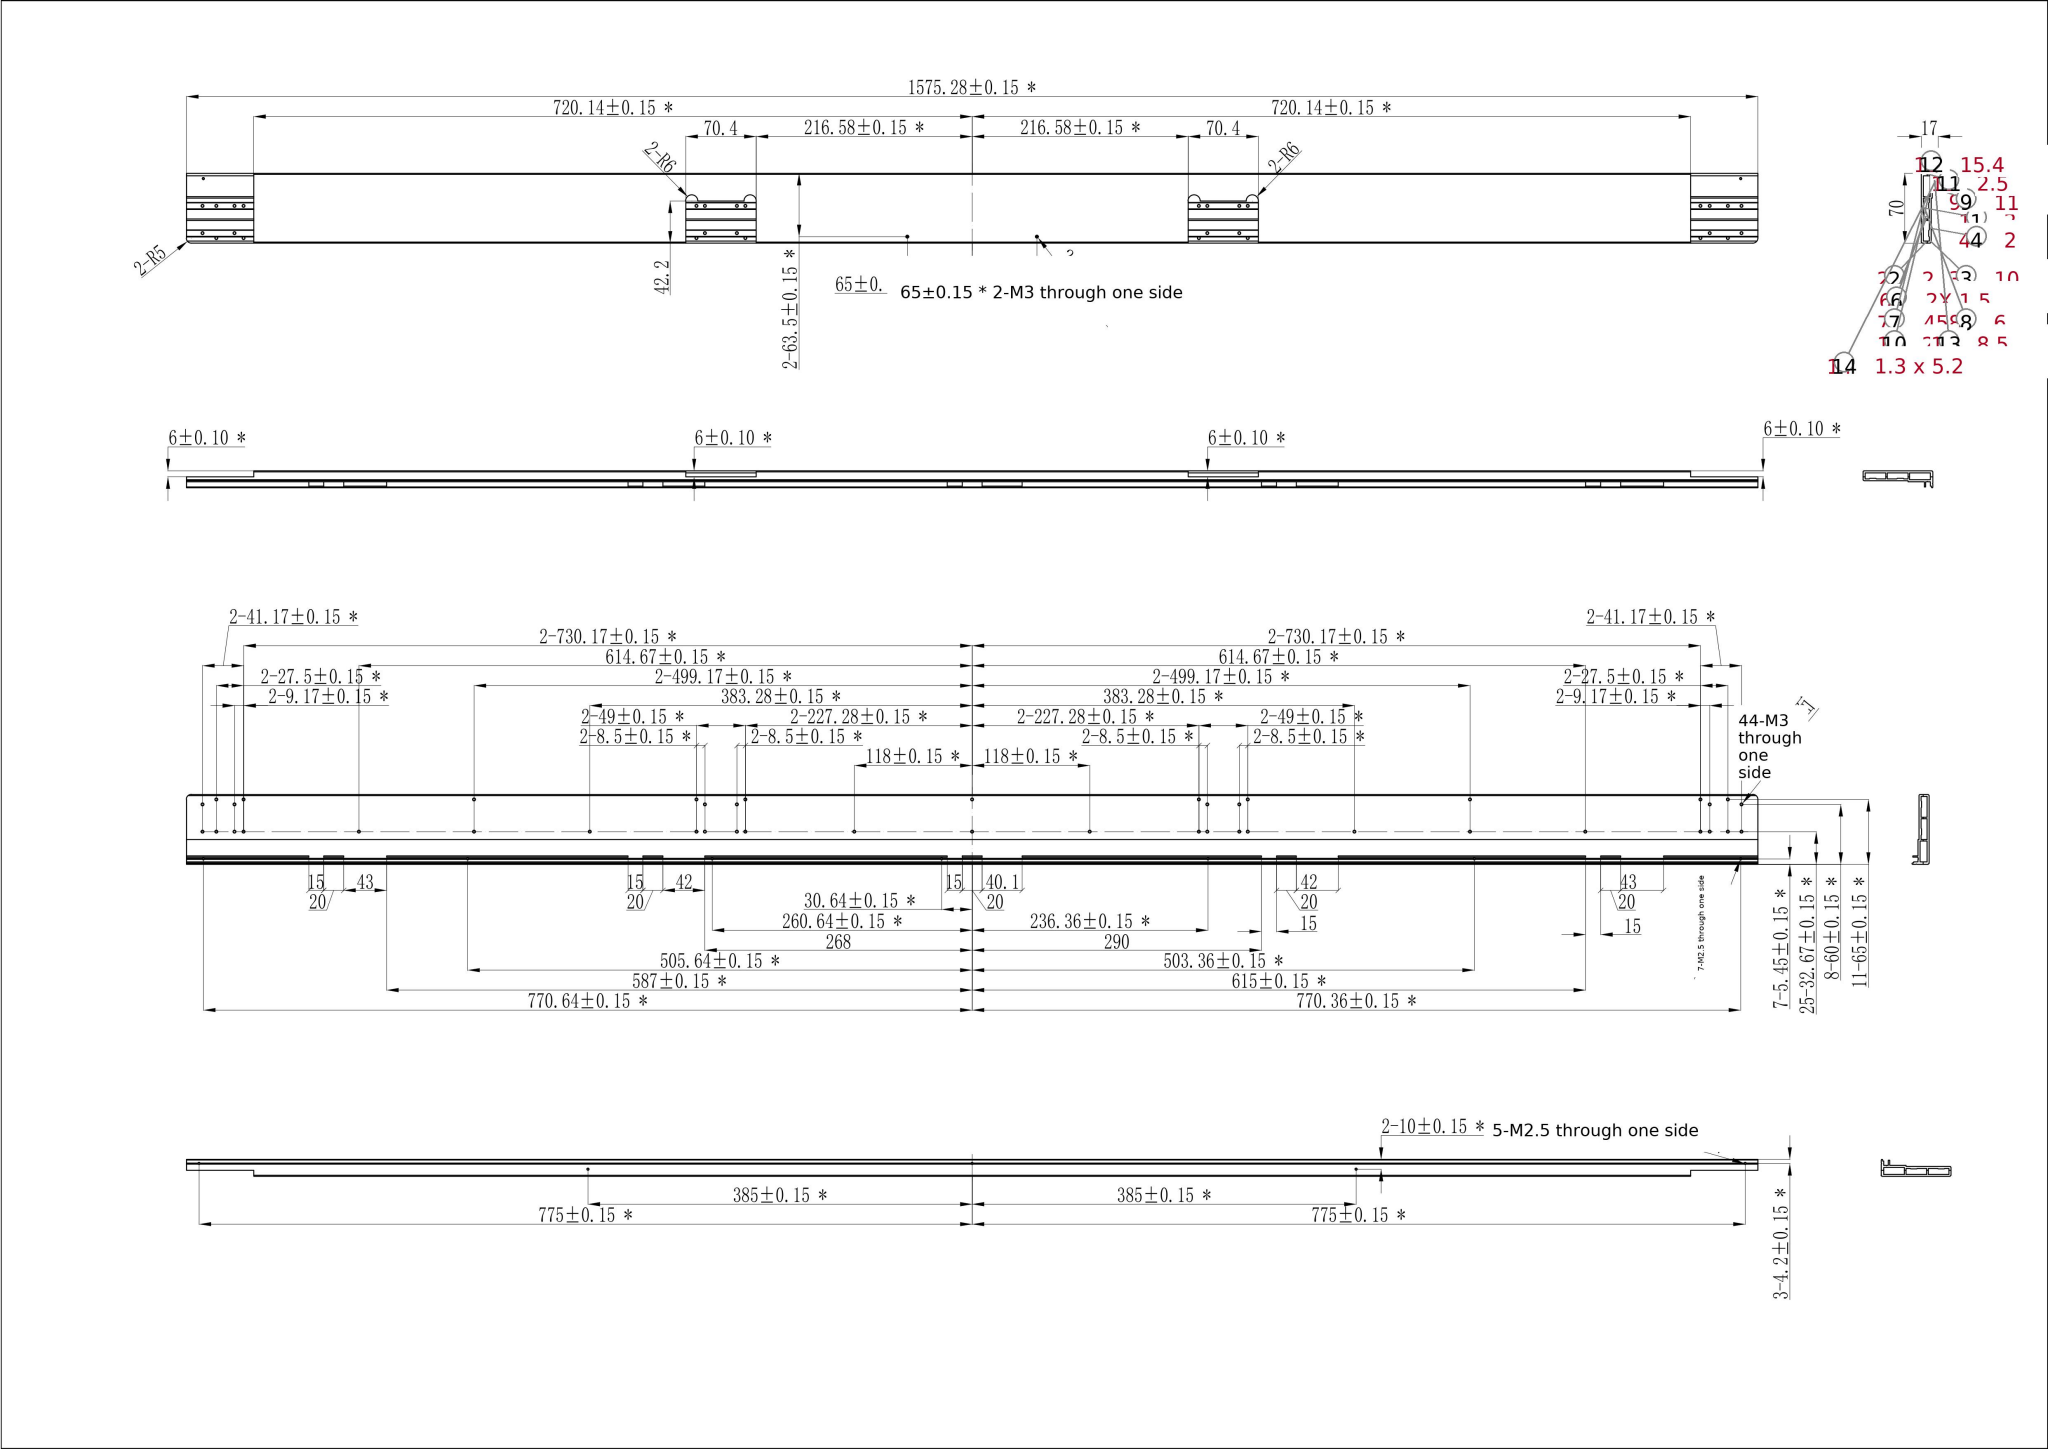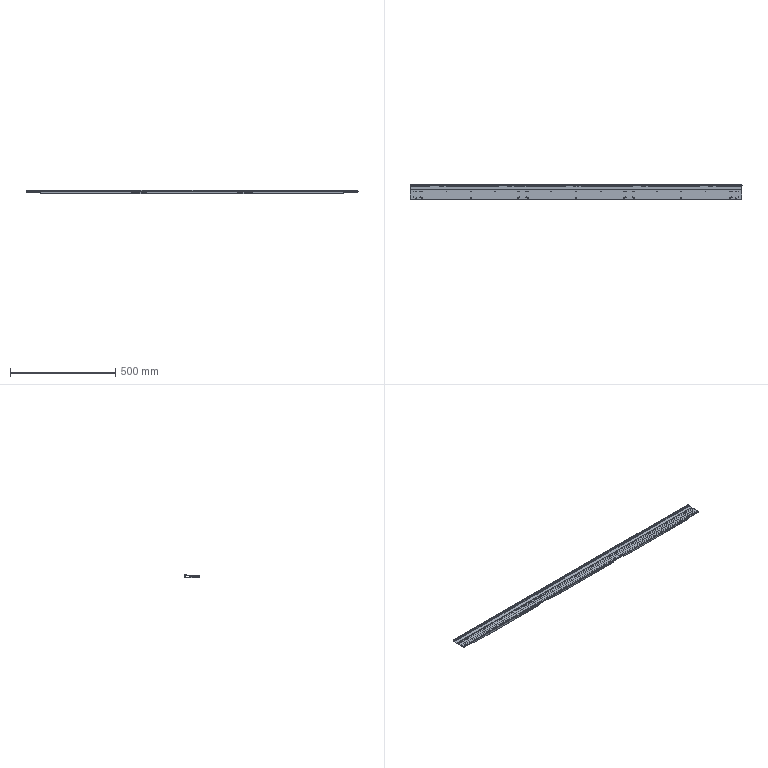Part | SolidWorks | mm | 1 solid | 361 faces | box 1575.28 x 70 x 17 mm | volume 518484 mm3 | plane 135 | cylinder 121 | cone 105 | commonest cylinder face diameters 3 x92 2.5 x24 2 x5